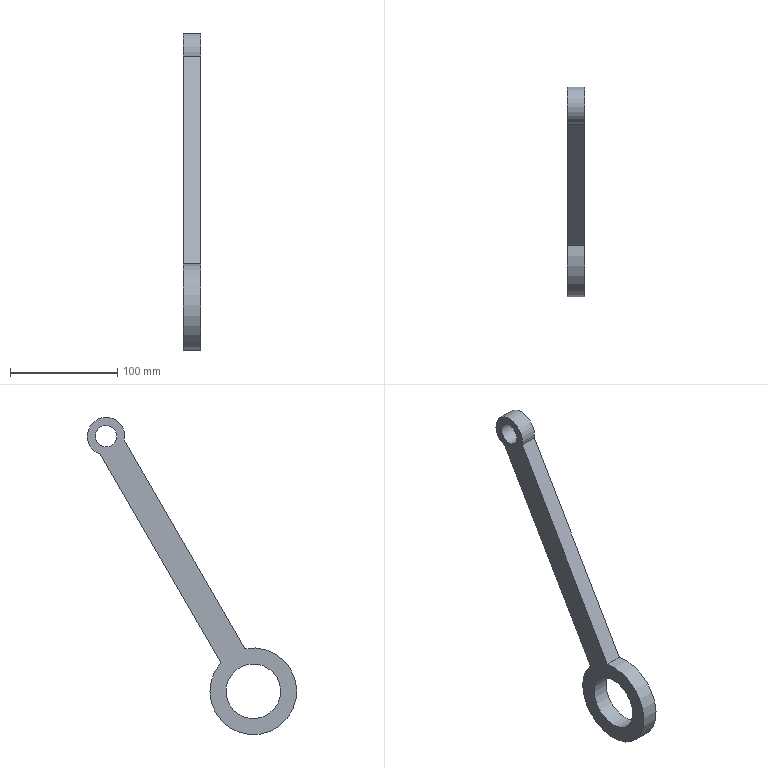Component | NX | CON_ROD_2 | 1 solid | 8 faces | box 15.9 x 195.5 x 296.16 mm | volume 150490 mm3 | cylinder 4 | plane 4 | commonest cylinder face diameters 81 x1 35 x1 20 x1 51 x1
STEP:
#1=CARTESIAN_POINT('',(0.,0.,0.));
#2=DIRECTION('',(0.,0.,1.));
#3=DIRECTION('',(1.,0.,0.));
#4=AXIS2_PLACEMENT_3D('',#1,#2,#3);
#5=CARTESIAN_POINT('',(46.,-40.32,127.313));
#6=VERTEX_POINT('',#5);
#7=CARTESIAN_POINT('',(46.,-17.804,114.313));
#8=VERTEX_POINT('',#7);
#9=CARTESIAN_POINT('',(46.,-48.24,87.595));
#10=DIRECTION('',(1.,0.,0.));
#11=DIRECTION('',(0.,0.866,-0.5));
#12=AXIS2_PLACEMENT_3D('',#9,#10,#11);
#13=CIRCLE('',#12,40.5);
#14=CARTESIAN_POINT('',(61.9,-48.24,87.595));
#15=DIRECTION('',(-1.,0.,0.));
#16=DIRECTION('',(0.,0.5,0.866));
#17=AXIS2_PLACEMENT_3D('',#14,#15,#16);
#18=CYLINDRICAL_SURFACE('',#17,40.5);
#19=CARTESIAN_POINT('',(7.854,15.9));
#20=DIRECTION('',(-1.,0.));
#21=VECTOR('',#20,1.);
#22=LINE('',#19,#21);
#23=(GEOMETRIC_REPRESENTATION_CONTEXT(2)PARAMETRIC_REPRESENTATION_CONTEXT()REPRESENTATION_CONTEXT('',''));
#24=DEFINITIONAL_REPRESENTATION('',(#22),#23);
#25=PCURVE('',#18,#24);
#26=CARTESIAN_POINT('',(46.,-48.24,87.595));
#27=DIRECTION('',(1.,0.,0.));
#28=DIRECTION('',(0.,-0.5,-0.866));
#29=AXIS2_PLACEMENT_3D('',#26,#27,#28);
#30=PLANE('',#29);
#31=CARTESIAN_POINT('',(0.,0.));
#32=DIRECTION('',(0.,1.));
#33=AXIS2_PLACEMENT_2D('',#31,#32);
#34=CIRCLE('',#33,40.5);
#35=(GEOMETRIC_REPRESENTATION_CONTEXT(2)PARAMETRIC_REPRESENTATION_CONTEXT()REPRESENTATION_CONTEXT('',''));
#36=DEFINITIONAL_REPRESENTATION('',(#34),#35);
#37=PCURVE('',#30,#36);
#38=SURFACE_CURVE('',#13,(#25,#37),.PCURVE_S1.);
#39=EDGE_CURVE('',#6,#8,#38,.T.);
#40=ORIENTED_EDGE('',*,*,#39,.T.);
#41=CARTESIAN_POINT('',(61.9,-17.804,114.313));
#42=VERTEX_POINT('',#41);
#43=CARTESIAN_POINT('',(61.9,-17.804,114.313));
#44=DIRECTION('',(-1.,0.,0.));
#45=VECTOR('',#44,1.);
#46=LINE('',#43,#45);
#47=CARTESIAN_POINT('',(0.3268,0.));
#48=DIRECTION('',(0.,1.));
#49=VECTOR('',#48,1.);
#50=LINE('',#47,#49);
#51=(GEOMETRIC_REPRESENTATION_CONTEXT(2)PARAMETRIC_REPRESENTATION_CONTEXT()REPRESENTATION_CONTEXT('',''));
#52=DEFINITIONAL_REPRESENTATION('',(#50),#51);
#53=PCURVE('',#18,#52);
#54=CARTESIAN_POINT('',(61.9,-17.804,114.313));
#55=DIRECTION('',(0.,-0.866,0.5));
#56=DIRECTION('',(0.,0.5,0.866));
#57=AXIS2_PLACEMENT_3D('',#54,#55,#56);
#58=PLANE('',#57);
#59=CARTESIAN_POINT('',(0.,0.));
#60=DIRECTION('',(0.,1.));
#61=VECTOR('',#60,1.);
#62=LINE('',#59,#61);
#63=(GEOMETRIC_REPRESENTATION_CONTEXT(2)PARAMETRIC_REPRESENTATION_CONTEXT()REPRESENTATION_CONTEXT('',''));
#64=DEFINITIONAL_REPRESENTATION('',(#62),#63);
#65=PCURVE('',#58,#64);
#66=SURFACE_CURVE('',#46,(#53,#65),.PCURVE_S1.);
#67=EDGE_CURVE('',#42,#8,#66,.T.);
#68=ORIENTED_EDGE('',*,*,#67,.F.);
#69=CARTESIAN_POINT('',(61.9,-40.32,127.313));
#70=VERTEX_POINT('',#69);
#71=CARTESIAN_POINT('',(61.9,-48.24,87.595));
#72=DIRECTION('',(1.,0.,0.));
#73=DIRECTION('',(0.,0.866,-0.5));
#74=AXIS2_PLACEMENT_3D('',#71,#72,#73);
#75=CIRCLE('',#74,40.5);
#76=CARTESIAN_POINT('',(7.854,0.));
#77=DIRECTION('',(-1.,0.));
#78=VECTOR('',#77,1.);
#79=LINE('',#76,#78);
#80=(GEOMETRIC_REPRESENTATION_CONTEXT(2)PARAMETRIC_REPRESENTATION_CONTEXT()REPRESENTATION_CONTEXT('',''));
#81=DEFINITIONAL_REPRESENTATION('',(#79),#80);
#82=PCURVE('',#18,#81);
#83=CARTESIAN_POINT('',(61.9,-48.24,87.595));
#84=DIRECTION('',(1.,0.,0.));
#85=DIRECTION('',(0.,-0.5,-0.866));
#86=AXIS2_PLACEMENT_3D('',#83,#84,#85);
#87=PLANE('',#86);
#88=CARTESIAN_POINT('',(0.,0.));
#89=DIRECTION('',(0.,1.));
#90=AXIS2_PLACEMENT_2D('',#88,#89);
#91=CIRCLE('',#90,40.5);
#92=(GEOMETRIC_REPRESENTATION_CONTEXT(2)PARAMETRIC_REPRESENTATION_CONTEXT()REPRESENTATION_CONTEXT('',''));
#93=DEFINITIONAL_REPRESENTATION('',(#91),#92);
#94=PCURVE('',#87,#93);
#95=SURFACE_CURVE('',#75,(#82,#94),.PCURVE_S1.);
#96=EDGE_CURVE('',#70,#42,#95,.T.);
#97=ORIENTED_EDGE('',*,*,#96,.F.);
#98=CARTESIAN_POINT('',(61.9,-40.32,127.313));
#99=DIRECTION('',(-1.,0.,0.));
#100=VECTOR('',#99,1.);
#101=LINE('',#98,#100);
#102=CARTESIAN_POINT('',(5.956,0.));
#103=DIRECTION('',(0.,1.));
#104=VECTOR('',#103,1.);
#105=LINE('',#102,#104);
#106=(GEOMETRIC_REPRESENTATION_CONTEXT(2)PARAMETRIC_REPRESENTATION_CONTEXT()REPRESENTATION_CONTEXT('',''));
#107=DEFINITIONAL_REPRESENTATION('',(#105),#106);
#108=PCURVE('',#18,#107);
#109=CARTESIAN_POINT('',(61.9,72.143,322.106));
#110=DIRECTION('',(0.,0.866,-0.5));
#111=DIRECTION('',(0.,-0.5,-0.866));
#112=AXIS2_PLACEMENT_3D('',#109,#110,#111);
#113=PLANE('',#112);
#114=CARTESIAN_POINT('',(224.928,0.));
#115=DIRECTION('',(0.,1.));
#116=VECTOR('',#115,1.);
#117=LINE('',#114,#116);
#118=(GEOMETRIC_REPRESENTATION_CONTEXT(2)PARAMETRIC_REPRESENTATION_CONTEXT()REPRESENTATION_CONTEXT('',''));
#119=DEFINITIONAL_REPRESENTATION('',(#117),#118);
#120=PCURVE('',#113,#119);
#121=SURFACE_CURVE('',#101,(#108,#120),.PCURVE_S1.);
#122=EDGE_CURVE('',#70,#6,#121,.T.);
#123=ORIENTED_EDGE('',*,*,#122,.T.);
#124=EDGE_LOOP('',(#40,#68,#97,#123));
#125=FACE_BOUND('',#124,.T.);
#126=ADVANCED_FACE('',(#125),#18,.T.);
#127=CARTESIAN_POINT('',(46.,94.66,309.106));
#128=VERTEX_POINT('',#127);
#129=CARTESIAN_POINT('',(46.,-17.804,114.313));
#130=DIRECTION('',(0.,0.5,0.866));
#131=VECTOR('',#130,1.);
#132=LINE('',#129,#131);
#133=CARTESIAN_POINT('',(0.,15.9));
#134=DIRECTION('',(1.,0.));
#135=VECTOR('',#134,1.);
#136=LINE('',#133,#135);
#137=(GEOMETRIC_REPRESENTATION_CONTEXT(2)PARAMETRIC_REPRESENTATION_CONTEXT()REPRESENTATION_CONTEXT('',''));
#138=DEFINITIONAL_REPRESENTATION('',(#136),#137);
#139=PCURVE('',#58,#138);
#140=CARTESIAN_POINT('',(-38.357,13.));
#141=DIRECTION('',(-1.,-0.));
#142=VECTOR('',#141,1.);
#143=LINE('',#140,#142);
#144=(GEOMETRIC_REPRESENTATION_CONTEXT(2)PARAMETRIC_REPRESENTATION_CONTEXT()REPRESENTATION_CONTEXT('',''));
#145=DEFINITIONAL_REPRESENTATION('',(#143),#144);
#146=PCURVE('',#30,#145);
#147=SURFACE_CURVE('',#132,(#139,#146),.PCURVE_S1.);
#148=EDGE_CURVE('',#8,#128,#147,.T.);
#149=ORIENTED_EDGE('',*,*,#148,.T.);
#150=CARTESIAN_POINT('',(61.9,94.66,309.106));
#151=VERTEX_POINT('',#150);
#152=CARTESIAN_POINT('',(61.9,94.66,309.106));
#153=DIRECTION('',(-1.,0.,0.));
#154=VECTOR('',#153,1.);
#155=LINE('',#152,#154);
#156=CARTESIAN_POINT('',(224.928,0.));
#157=DIRECTION('',(0.,1.));
#158=VECTOR('',#157,1.);
#159=LINE('',#156,#158);
#160=(GEOMETRIC_REPRESENTATION_CONTEXT(2)PARAMETRIC_REPRESENTATION_CONTEXT()REPRESENTATION_CONTEXT('',''));
#161=DEFINITIONAL_REPRESENTATION('',(#159),#160);
#162=PCURVE('',#58,#161);
#163=CARTESIAN_POINT('',(61.9,89.26,325.752));
#164=DIRECTION('',(-1.,0.,0.));
#165=DIRECTION('',(0.,0.5,0.866));
#166=AXIS2_PLACEMENT_3D('',#163,#164,#165);
#167=CYLINDRICAL_SURFACE('',#166,17.5);
#168=CARTESIAN_POINT('',(2.304,0.));
#169=DIRECTION('',(0.,1.));
#170=VECTOR('',#169,1.);
#171=LINE('',#168,#170);
#172=(GEOMETRIC_REPRESENTATION_CONTEXT(2)PARAMETRIC_REPRESENTATION_CONTEXT()REPRESENTATION_CONTEXT('',''));
#173=DEFINITIONAL_REPRESENTATION('',(#171),#172);
#174=PCURVE('',#167,#173);
#175=SURFACE_CURVE('',#155,(#162,#174),.PCURVE_S1.);
#176=EDGE_CURVE('',#151,#128,#175,.T.);
#177=ORIENTED_EDGE('',*,*,#176,.F.);
#178=CARTESIAN_POINT('',(61.9,-17.804,114.313));
#179=DIRECTION('',(0.,0.5,0.866));
#180=VECTOR('',#179,1.);
#181=LINE('',#178,#180);
#182=CARTESIAN_POINT('',(0.,0.));
#183=DIRECTION('',(1.,0.));
#184=VECTOR('',#183,1.);
#185=LINE('',#182,#184);
#186=(GEOMETRIC_REPRESENTATION_CONTEXT(2)PARAMETRIC_REPRESENTATION_CONTEXT()REPRESENTATION_CONTEXT('',''));
#187=DEFINITIONAL_REPRESENTATION('',(#185),#186);
#188=PCURVE('',#58,#187);
#189=CARTESIAN_POINT('',(-38.357,13.));
#190=DIRECTION('',(-1.,-0.));
#191=VECTOR('',#190,1.);
#192=LINE('',#189,#191);
#193=(GEOMETRIC_REPRESENTATION_CONTEXT(2)PARAMETRIC_REPRESENTATION_CONTEXT()REPRESENTATION_CONTEXT('',''));
#194=DEFINITIONAL_REPRESENTATION('',(#192),#193);
#195=PCURVE('',#87,#194);
#196=SURFACE_CURVE('',#181,(#188,#195),.PCURVE_S1.);
#197=EDGE_CURVE('',#42,#151,#196,.T.);
#198=ORIENTED_EDGE('',*,*,#197,.F.);
#199=ORIENTED_EDGE('',*,*,#67,.T.);
#200=EDGE_LOOP('',(#149,#177,#198,#199));
#201=FACE_BOUND('',#200,.T.);
#202=ADVANCED_FACE('',(#201),#58,.F.);
#203=CARTESIAN_POINT('',(46.,72.143,322.106));
#204=VERTEX_POINT('',#203);
#205=CARTESIAN_POINT('',(46.,89.26,325.752));
#206=DIRECTION('',(1.,0.,0.));
#207=DIRECTION('',(0.,0.866,-0.5));
#208=AXIS2_PLACEMENT_3D('',#205,#206,#207);
#209=CIRCLE('',#208,17.5);
#210=CARTESIAN_POINT('',(7.854,15.9));
#211=DIRECTION('',(-1.,0.));
#212=VECTOR('',#211,1.);
#213=LINE('',#210,#212);
#214=(GEOMETRIC_REPRESENTATION_CONTEXT(2)PARAMETRIC_REPRESENTATION_CONTEXT()REPRESENTATION_CONTEXT('',''));
#215=DEFINITIONAL_REPRESENTATION('',(#213),#214);
#216=PCURVE('',#167,#215);
#217=CARTESIAN_POINT('',(-275.,-0.));
#218=DIRECTION('',(0.,1.));
#219=AXIS2_PLACEMENT_2D('',#217,#218);
#220=CIRCLE('',#219,17.5);
#221=(GEOMETRIC_REPRESENTATION_CONTEXT(2)PARAMETRIC_REPRESENTATION_CONTEXT()REPRESENTATION_CONTEXT('',''));
#222=DEFINITIONAL_REPRESENTATION('',(#220),#221);
#223=PCURVE('',#30,#222);
#224=SURFACE_CURVE('',#209,(#216,#223),.PCURVE_S1.);
#225=EDGE_CURVE('',#128,#204,#224,.T.);
#226=ORIENTED_EDGE('',*,*,#225,.T.);
#227=CARTESIAN_POINT('',(61.9,72.143,322.106));
#228=VERTEX_POINT('',#227);
#229=CARTESIAN_POINT('',(61.9,72.143,322.106));
#230=DIRECTION('',(-1.,0.,0.));
#231=VECTOR('',#230,1.);
#232=LINE('',#229,#231);
#233=CARTESIAN_POINT('',(-2.304,0.));
#234=DIRECTION('',(0.,1.));
#235=VECTOR('',#234,1.);
#236=LINE('',#233,#235);
#237=(GEOMETRIC_REPRESENTATION_CONTEXT(2)PARAMETRIC_REPRESENTATION_CONTEXT()REPRESENTATION_CONTEXT('',''));
#238=DEFINITIONAL_REPRESENTATION('',(#236),#237);
#239=PCURVE('',#167,#238);
#240=CARTESIAN_POINT('',(0.,0.));
#241=DIRECTION('',(0.,1.));
#242=VECTOR('',#241,1.);
#243=LINE('',#240,#242);
#244=(GEOMETRIC_REPRESENTATION_CONTEXT(2)PARAMETRIC_REPRESENTATION_CONTEXT()REPRESENTATION_CONTEXT('',''));
#245=DEFINITIONAL_REPRESENTATION('',(#243),#244);
#246=PCURVE('',#113,#245);
#247=SURFACE_CURVE('',#232,(#239,#246),.PCURVE_S1.);
#248=EDGE_CURVE('',#228,#204,#247,.T.);
#249=ORIENTED_EDGE('',*,*,#248,.F.);
#250=CARTESIAN_POINT('',(61.9,89.26,325.752));
#251=DIRECTION('',(1.,0.,0.));
#252=DIRECTION('',(0.,0.866,-0.5));
#253=AXIS2_PLACEMENT_3D('',#250,#251,#252);
#254=CIRCLE('',#253,17.5);
#255=CARTESIAN_POINT('',(7.854,0.));
#256=DIRECTION('',(-1.,0.));
#257=VECTOR('',#256,1.);
#258=LINE('',#255,#257);
#259=(GEOMETRIC_REPRESENTATION_CONTEXT(2)PARAMETRIC_REPRESENTATION_CONTEXT()REPRESENTATION_CONTEXT('',''));
#260=DEFINITIONAL_REPRESENTATION('',(#258),#259);
#261=PCURVE('',#167,#260);
#262=CARTESIAN_POINT('',(-275.,-0.));
#263=DIRECTION('',(0.,1.));
#264=AXIS2_PLACEMENT_2D('',#262,#263);
#265=CIRCLE('',#264,17.5);
#266=(GEOMETRIC_REPRESENTATION_CONTEXT(2)PARAMETRIC_REPRESENTATION_CONTEXT()REPRESENTATION_CONTEXT('',''));
#267=DEFINITIONAL_REPRESENTATION('',(#265),#266);
#268=PCURVE('',#87,#267);
#269=SURFACE_CURVE('',#254,(#261,#268),.PCURVE_S1.);
#270=EDGE_CURVE('',#151,#228,#269,.T.);
#271=ORIENTED_EDGE('',*,*,#270,.F.);
#272=ORIENTED_EDGE('',*,*,#176,.T.);
#273=EDGE_LOOP('',(#226,#249,#271,#272));
#274=FACE_BOUND('',#273,.T.);
#275=ADVANCED_FACE('',(#274),#167,.T.);
#276=CARTESIAN_POINT('',(61.9,97.92,320.752));
#277=VERTEX_POINT('',#276);
#278=CARTESIAN_POINT('',(61.9,89.26,325.752));
#279=DIRECTION('',(1.,0.,0.));
#280=DIRECTION('',(0.,0.866,-0.5));
#281=AXIS2_PLACEMENT_3D('',#278,#279,#280);
#282=CIRCLE('',#281,10.);
#283=CARTESIAN_POINT('',(61.9,89.26,325.752));
#284=DIRECTION('',(-1.,0.,0.));
#285=DIRECTION('',(0.,0.5,0.866));
#286=AXIS2_PLACEMENT_3D('',#283,#284,#285);
#287=CYLINDRICAL_SURFACE('',#286,10.);
#288=CARTESIAN_POINT('',(7.854,0.));
#289=DIRECTION('',(-1.,0.));
#290=VECTOR('',#289,1.);
#291=LINE('',#288,#290);
#292=(GEOMETRIC_REPRESENTATION_CONTEXT(2)PARAMETRIC_REPRESENTATION_CONTEXT()REPRESENTATION_CONTEXT('',''));
#293=DEFINITIONAL_REPRESENTATION('',(#291),#292);
#294=PCURVE('',#287,#293);
#295=CARTESIAN_POINT('',(-275.,-0.));
#296=DIRECTION('',(0.,1.));
#297=AXIS2_PLACEMENT_2D('',#295,#296);
#298=CIRCLE('',#297,10.);
#299=(GEOMETRIC_REPRESENTATION_CONTEXT(2)PARAMETRIC_REPRESENTATION_CONTEXT()REPRESENTATION_CONTEXT('',''));
#300=DEFINITIONAL_REPRESENTATION('',(#298),#299);
#301=PCURVE('',#87,#300);
#302=SURFACE_CURVE('',#282,(#294,#301),.PCURVE_S1.);
#303=EDGE_CURVE('',#277,#277,#302,.T.);
#304=ORIENTED_EDGE('',*,*,#303,.F.);
#305=CARTESIAN_POINT('',(46.,97.92,320.752));
#306=VERTEX_POINT('',#305);
#307=CARTESIAN_POINT('',(61.9,97.92,320.752));
#308=CARTESIAN_POINT('',(46.,97.92,320.752));
#309=B_SPLINE_CURVE_WITH_KNOTS('',1,(#307,#308),.UNSPECIFIED.,.F.,.F.,(2,2),(0.,15.9),.PIECEWISE_BEZIER_KNOTS.);
#310=CARTESIAN_POINT('',(7.854,0.));
#311=DIRECTION('',(0.,1.));
#312=VECTOR('',#311,1.);
#313=LINE('',#310,#312);
#314=(GEOMETRIC_REPRESENTATION_CONTEXT(2)PARAMETRIC_REPRESENTATION_CONTEXT()REPRESENTATION_CONTEXT('',''));
#315=DEFINITIONAL_REPRESENTATION('',(#313),#314);
#316=PCURVE('',#287,#315);
#317=CARTESIAN_POINT('',(1.571,0.));
#318=DIRECTION('',(0.,1.));
#319=VECTOR('',#318,1.);
#320=LINE('',#317,#319);
#321=(GEOMETRIC_REPRESENTATION_CONTEXT(2)PARAMETRIC_REPRESENTATION_CONTEXT()REPRESENTATION_CONTEXT('',''));
#322=DEFINITIONAL_REPRESENTATION('',(#320),#321);
#323=PCURVE('',#287,#322);
#324=SEAM_CURVE('',#309,(#316,#323),.PCURVE_S1.);
#325=EDGE_CURVE('',#277,#306,#324,.T.);
#326=ORIENTED_EDGE('',*,*,#325,.T.);
#327=CARTESIAN_POINT('',(46.,89.26,325.752));
#328=DIRECTION('',(1.,0.,0.));
#329=DIRECTION('',(0.,0.866,-0.5));
#330=AXIS2_PLACEMENT_3D('',#327,#328,#329);
#331=CIRCLE('',#330,10.);
#332=CARTESIAN_POINT('',(7.854,15.9));
#333=DIRECTION('',(-1.,0.));
#334=VECTOR('',#333,1.);
#335=LINE('',#332,#334);
#336=(GEOMETRIC_REPRESENTATION_CONTEXT(2)PARAMETRIC_REPRESENTATION_CONTEXT()REPRESENTATION_CONTEXT('',''));
#337=DEFINITIONAL_REPRESENTATION('',(#335),#336);
#338=PCURVE('',#287,#337);
#339=CARTESIAN_POINT('',(-275.,-0.));
#340=DIRECTION('',(0.,1.));
#341=AXIS2_PLACEMENT_2D('',#339,#340);
#342=CIRCLE('',#341,10.);
#343=(GEOMETRIC_REPRESENTATION_CONTEXT(2)PARAMETRIC_REPRESENTATION_CONTEXT()REPRESENTATION_CONTEXT('',''));
#344=DEFINITIONAL_REPRESENTATION('',(#342),#343);
#345=PCURVE('',#30,#344);
#346=SURFACE_CURVE('',#331,(#338,#345),.PCURVE_S1.);
#347=EDGE_CURVE('',#306,#306,#346,.T.);
#348=ORIENTED_EDGE('',*,*,#347,.T.);
#349=ORIENTED_EDGE('',*,*,#325,.F.);
#350=EDGE_LOOP('',(#304,#326,#348,#349));
#351=FACE_BOUND('',#350,.F.);
#352=ADVANCED_FACE('',(#351),#287,.F.);
#353=CARTESIAN_POINT('',(46.,72.143,322.106));
#354=DIRECTION('',(0.,-0.5,-0.866));
#355=VECTOR('',#354,1.);
#356=LINE('',#353,#355);
#357=CARTESIAN_POINT('',(0.,15.9));
#358=DIRECTION('',(1.,0.));
#359=VECTOR('',#358,1.);
#360=LINE('',#357,#359);
#361=(GEOMETRIC_REPRESENTATION_CONTEXT(2)PARAMETRIC_REPRESENTATION_CONTEXT()REPRESENTATION_CONTEXT('',''));
#362=DEFINITIONAL_REPRESENTATION('',(#360),#361);
#363=PCURVE('',#113,#362);
#364=CARTESIAN_POINT('',(-263.285,-13.));
#365=DIRECTION('',(1.,-0.));
#366=VECTOR('',#365,1.);
#367=LINE('',#364,#366);
#368=(GEOMETRIC_REPRESENTATION_CONTEXT(2)PARAMETRIC_REPRESENTATION_CONTEXT()REPRESENTATION_CONTEXT('',''));
#369=DEFINITIONAL_REPRESENTATION('',(#367),#368);
#370=PCURVE('',#30,#369);
#371=SURFACE_CURVE('',#356,(#363,#370),.PCURVE_S1.);
#372=EDGE_CURVE('',#204,#6,#371,.T.);
#373=ORIENTED_EDGE('',*,*,#372,.T.);
#374=ORIENTED_EDGE('',*,*,#122,.F.);
#375=CARTESIAN_POINT('',(61.9,72.143,322.106));
#376=DIRECTION('',(0.,-0.5,-0.866));
#377=VECTOR('',#376,1.);
#378=LINE('',#375,#377);
#379=CARTESIAN_POINT('',(0.,0.));
#380=DIRECTION('',(1.,0.));
#381=VECTOR('',#380,1.);
#382=LINE('',#379,#381);
#383=(GEOMETRIC_REPRESENTATION_CONTEXT(2)PARAMETRIC_REPRESENTATION_CONTEXT()REPRESENTATION_CONTEXT('',''));
#384=DEFINITIONAL_REPRESENTATION('',(#382),#383);
#385=PCURVE('',#113,#384);
#386=CARTESIAN_POINT('',(-263.285,-13.));
#387=DIRECTION('',(1.,-0.));
#388=VECTOR('',#387,1.);
#389=LINE('',#386,#388);
#390=(GEOMETRIC_REPRESENTATION_CONTEXT(2)PARAMETRIC_REPRESENTATION_CONTEXT()REPRESENTATION_CONTEXT('',''));
#391=DEFINITIONAL_REPRESENTATION('',(#389),#390);
#392=PCURVE('',#87,#391);
#393=SURFACE_CURVE('',#378,(#385,#392),.PCURVE_S1.);
#394=EDGE_CURVE('',#228,#70,#393,.T.);
#395=ORIENTED_EDGE('',*,*,#394,.F.);
#396=ORIENTED_EDGE('',*,*,#248,.T.);
#397=EDGE_LOOP('',(#373,#374,#395,#396));
#398=FACE_BOUND('',#397,.T.);
#399=ADVANCED_FACE('',(#398),#113,.F.);
#400=CARTESIAN_POINT('',(61.9,-26.157,74.845));
#401=VERTEX_POINT('',#400);
#402=CARTESIAN_POINT('',(61.9,-48.24,87.595));
#403=DIRECTION('',(1.,0.,0.));
#404=DIRECTION('',(0.,0.866,-0.5));
#405=AXIS2_PLACEMENT_3D('',#402,#403,#404);
#406=CIRCLE('',#405,25.5);
#407=CARTESIAN_POINT('',(61.9,-48.24,87.595));
#408=DIRECTION('',(-1.,0.,0.));
#409=DIRECTION('',(0.,0.5,0.866));
#410=AXIS2_PLACEMENT_3D('',#407,#408,#409);
#411=CYLINDRICAL_SURFACE('',#410,25.5);
#412=CARTESIAN_POINT('',(7.854,0.));
#413=DIRECTION('',(-1.,0.));
#414=VECTOR('',#413,1.);
#415=LINE('',#412,#414);
#416=(GEOMETRIC_REPRESENTATION_CONTEXT(2)PARAMETRIC_REPRESENTATION_CONTEXT()REPRESENTATION_CONTEXT('',''));
#417=DEFINITIONAL_REPRESENTATION('',(#415),#416);
#418=PCURVE('',#411,#417);
#419=CARTESIAN_POINT('',(0.,0.));
#420=DIRECTION('',(0.,1.));
#421=AXIS2_PLACEMENT_2D('',#419,#420);
#422=CIRCLE('',#421,25.5);
#423=(GEOMETRIC_REPRESENTATION_CONTEXT(2)PARAMETRIC_REPRESENTATION_CONTEXT()REPRESENTATION_CONTEXT('',''));
#424=DEFINITIONAL_REPRESENTATION('',(#422),#423);
#425=PCURVE('',#87,#424);
#426=SURFACE_CURVE('',#406,(#418,#425),.PCURVE_S1.);
#427=EDGE_CURVE('',#401,#401,#426,.T.);
#428=ORIENTED_EDGE('',*,*,#427,.F.);
#429=CARTESIAN_POINT('',(46.,-26.157,74.845));
#430=VERTEX_POINT('',#429);
#431=CARTESIAN_POINT('',(61.9,-26.157,74.845));
#432=CARTESIAN_POINT('',(46.,-26.157,74.845));
#433=B_SPLINE_CURVE_WITH_KNOTS('',1,(#431,#432),.UNSPECIFIED.,.F.,.F.,(2,2),(0.,15.9),.PIECEWISE_BEZIER_KNOTS.);
#434=CARTESIAN_POINT('',(7.854,0.));
#435=DIRECTION('',(0.,1.));
#436=VECTOR('',#435,1.);
#437=LINE('',#434,#436);
#438=(GEOMETRIC_REPRESENTATION_CONTEXT(2)PARAMETRIC_REPRESENTATION_CONTEXT()REPRESENTATION_CONTEXT('',''));
#439=DEFINITIONAL_REPRESENTATION('',(#437),#438);
#440=PCURVE('',#411,#439);
#441=CARTESIAN_POINT('',(1.571,0.));
#442=DIRECTION('',(0.,1.));
#443=VECTOR('',#442,1.);
#444=LINE('',#441,#443);
#445=(GEOMETRIC_REPRESENTATION_CONTEXT(2)PARAMETRIC_REPRESENTATION_CONTEXT()REPRESENTATION_CONTEXT('',''));
#446=DEFINITIONAL_REPRESENTATION('',(#444),#445);
#447=PCURVE('',#411,#446);
#448=SEAM_CURVE('',#433,(#440,#447),.PCURVE_S1.);
#449=EDGE_CURVE('',#401,#430,#448,.T.);
#450=ORIENTED_EDGE('',*,*,#449,.T.);
#451=CARTESIAN_POINT('',(46.,-48.24,87.595));
#452=DIRECTION('',(1.,0.,0.));
#453=DIRECTION('',(0.,0.866,-0.5));
#454=AXIS2_PLACEMENT_3D('',#451,#452,#453);
#455=CIRCLE('',#454,25.5);
#456=CARTESIAN_POINT('',(7.854,15.9));
#457=DIRECTION('',(-1.,0.));
#458=VECTOR('',#457,1.);
#459=LINE('',#456,#458);
#460=(GEOMETRIC_REPRESENTATION_CONTEXT(2)PARAMETRIC_REPRESENTATION_CONTEXT()REPRESENTATION_CONTEXT('',''));
#461=DEFINITIONAL_REPRESENTATION('',(#459),#460);
#462=PCURVE('',#411,#461);
#463=CARTESIAN_POINT('',(0.,0.));
#464=DIRECTION('',(0.,1.));
#465=AXIS2_PLACEMENT_2D('',#463,#464);
#466=CIRCLE('',#465,25.5);
#467=(GEOMETRIC_REPRESENTATION_CONTEXT(2)PARAMETRIC_REPRESENTATION_CONTEXT()REPRESENTATION_CONTEXT('',''));
#468=DEFINITIONAL_REPRESENTATION('',(#466),#467);
#469=PCURVE('',#30,#468);
#470=SURFACE_CURVE('',#455,(#462,#469),.PCURVE_S1.);
#471=EDGE_CURVE('',#430,#430,#470,.T.);
#472=ORIENTED_EDGE('',*,*,#471,.T.);
#473=ORIENTED_EDGE('',*,*,#449,.F.);
#474=EDGE_LOOP('',(#428,#450,#472,#473));
#475=FACE_BOUND('',#474,.F.);
#476=ADVANCED_FACE('',(#475),#411,.F.);
#477=ORIENTED_EDGE('',*,*,#96,.T.);
#478=ORIENTED_EDGE('',*,*,#197,.T.);
#479=ORIENTED_EDGE('',*,*,#270,.T.);
#480=ORIENTED_EDGE('',*,*,#394,.T.);
#481=EDGE_LOOP('',(#477,#478,#479,#480));
#482=FACE_BOUND('',#481,.T.);
#483=ORIENTED_EDGE('',*,*,#303,.F.);
#484=EDGE_LOOP('',(#483));
#485=FACE_BOUND('',#484,.T.);
#486=ORIENTED_EDGE('',*,*,#427,.F.);
#487=EDGE_LOOP('',(#486));
#488=FACE_BOUND('',#487,.T.);
#489=ADVANCED_FACE('',(#482,#485,#488),#87,.T.);
#490=ORIENTED_EDGE('',*,*,#39,.F.);
#491=ORIENTED_EDGE('',*,*,#372,.F.);
#492=ORIENTED_EDGE('',*,*,#225,.F.);
#493=ORIENTED_EDGE('',*,*,#148,.F.);
#494=EDGE_LOOP('',(#490,#491,#492,#493));
#495=FACE_BOUND('',#494,.T.);
#496=ORIENTED_EDGE('',*,*,#347,.T.);
#497=EDGE_LOOP('',(#496));
#498=FACE_BOUND('',#497,.T.);
#499=ORIENTED_EDGE('',*,*,#471,.T.);
#500=EDGE_LOOP('',(#499));
#501=FACE_BOUND('',#500,.T.);
#502=ADVANCED_FACE('',(#495,#498,#501),#30,.F.);
#503=CLOSED_SHELL('',(#126,#202,#275,#352,#399,#476,#489,#502));
#504=MANIFOLD_SOLID_BREP('',#503);
#505=(LENGTH_UNIT()NAMED_UNIT(*)SI_UNIT(.MILLI.,.METRE.));
#506=UNCERTAINTY_MEASURE_WITH_UNIT(LENGTH_MEASURE(0.000002),#505,'','');
#507=(NAMED_UNIT(*)PLANE_ANGLE_UNIT()SI_UNIT($,.RADIAN.));
#508=(NAMED_UNIT(*)SI_UNIT($,.STERADIAN.)SOLID_ANGLE_UNIT());
#509=(GEOMETRIC_REPRESENTATION_CONTEXT(3)GLOBAL_UNCERTAINTY_ASSIGNED_CONTEXT((#506))GLOBAL_UNIT_ASSIGNED_CONTEXT((#505,#507,#508))REPRESENTATION_CONTEXT('',''));
#510=ADVANCED_BREP_SHAPE_REPRESENTATION('',(#4,#504),#509);